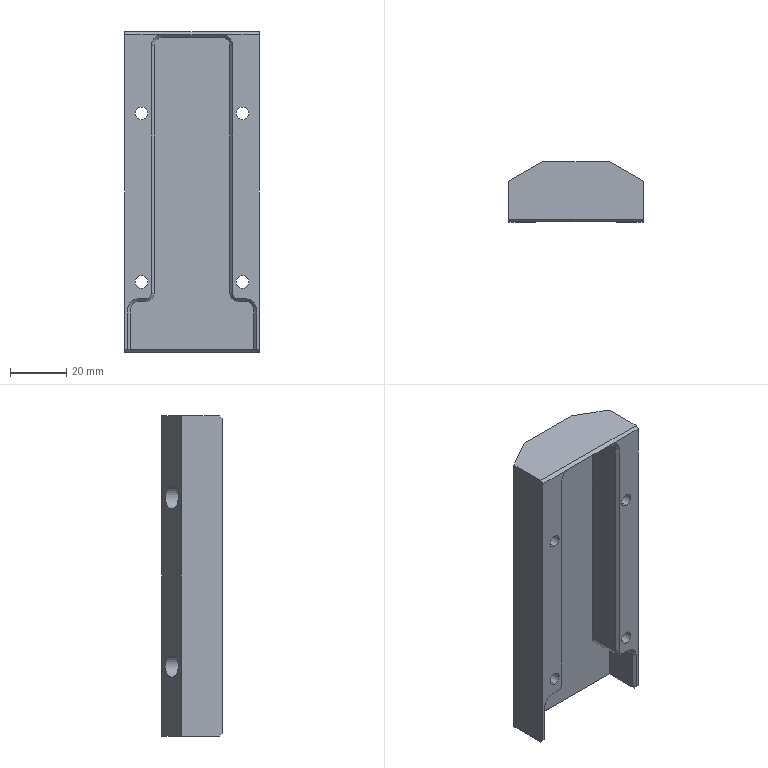CAM job | Mastercam | mm | 17 operations | part box 48 x 21.5 x 114
1. Contour (Ramp) | 9 - 10C 平底刀
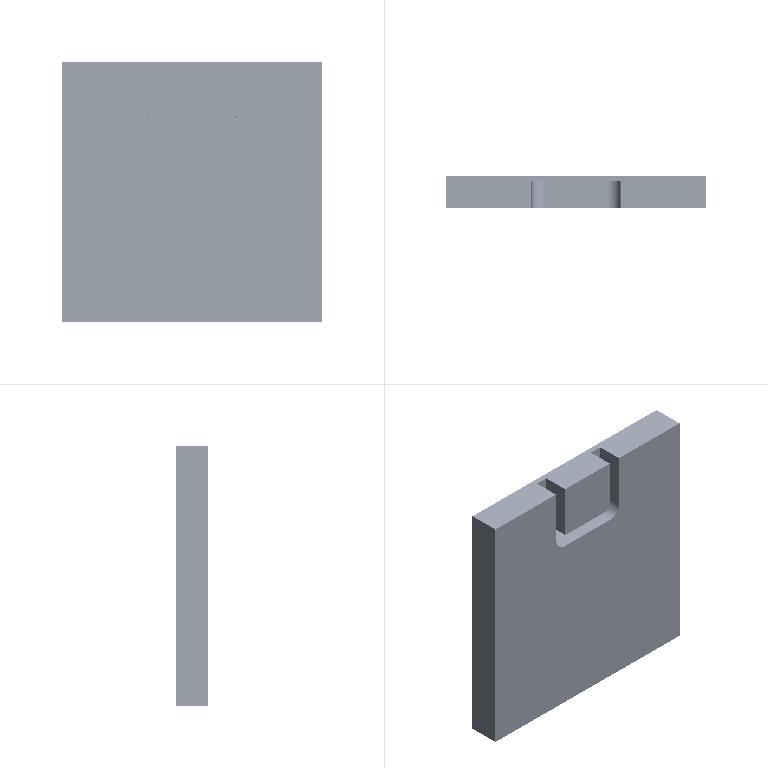2. Facing | 10 - 10J 平底刀
3. 2D High Speed (2D Dynamic Mill) | 6 - 6 平底刀
4. Drill/Counterbore | 2 - 4定位倒角
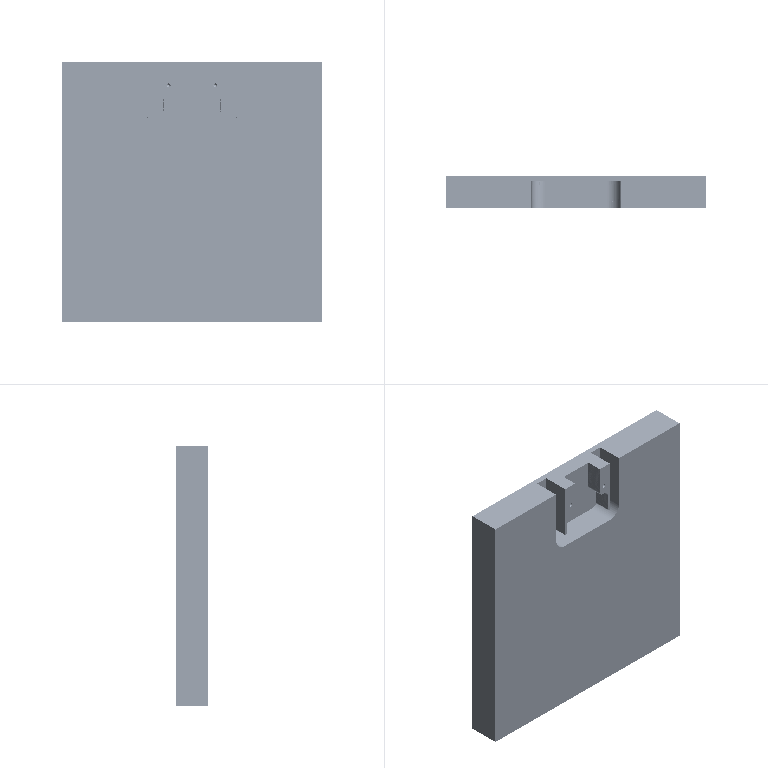5. Peck Drill | 18 - 4.5 钻头
6. Pocket (Open) | 8 - 6 J平底刀
7. Contour (2D) | 6 - 6 平底刀
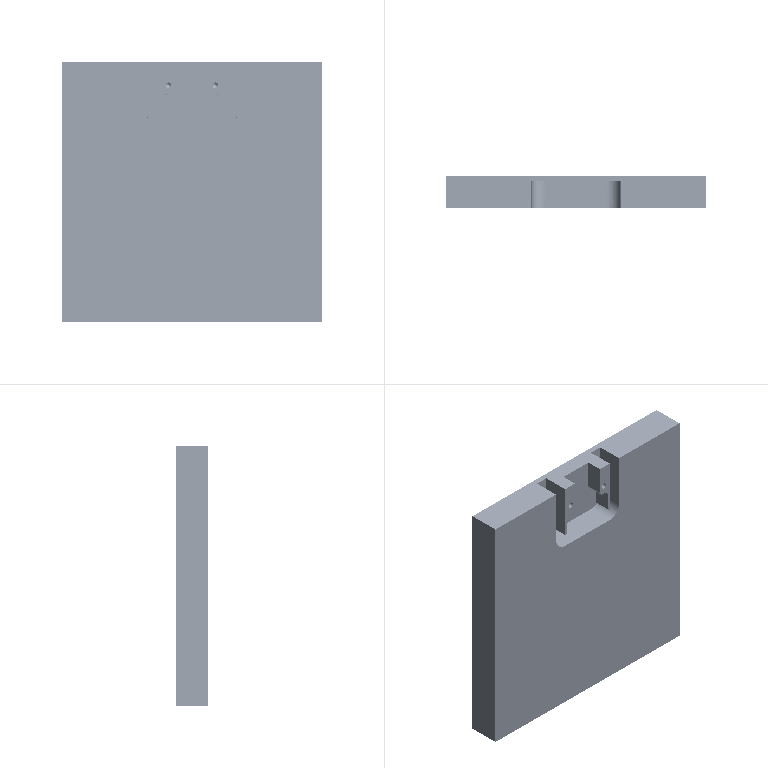8. Contour (2D chamfer) | 2 - 4定位倒角
9. Model Chamfer | 2 - 4定位倒角
10. Surface Finish Flowline | 20 - 4 -R0.5圆鼻铣刀
11. Contour (Ramp) | 9 - 10C 平底刀
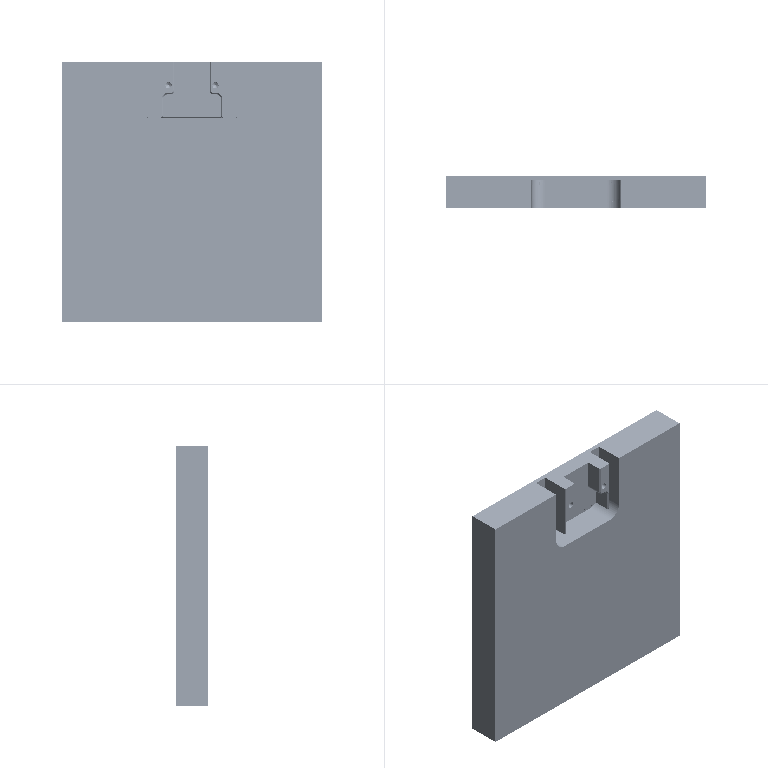12. Contour (2D) | 10 - 10J 平底刀
13. Facing | 1 - 50 J面铣
14. Helix Bore | 6 - 6 平底刀
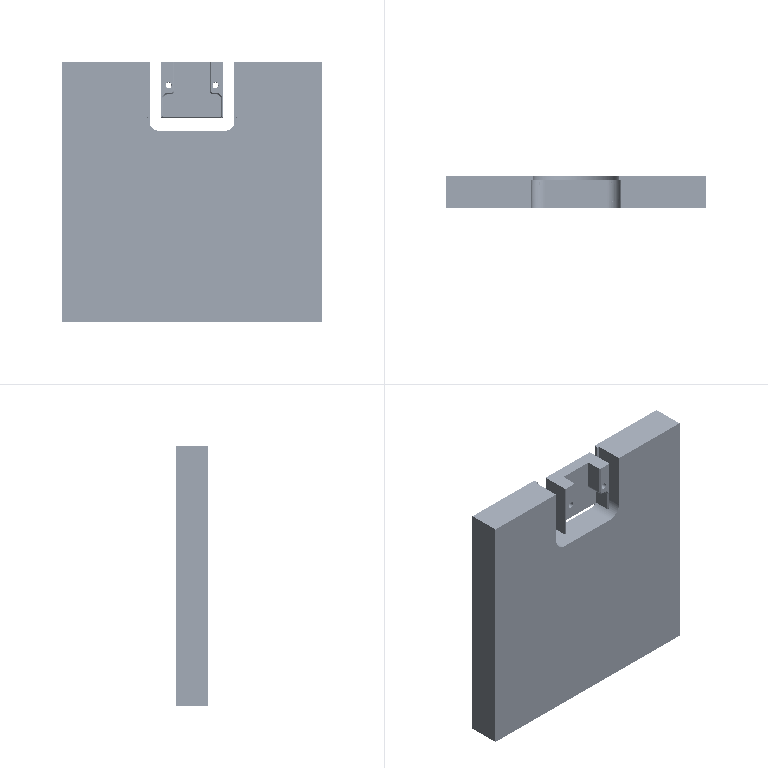15. Surface Finish Flowline | 3 - 10 -R1.0圆鼻铣刀
16. Deburr 5-axis Deburr 5-axis | 24 - 4 球刀
17. Contour (Ramp) | 9 - 10C 平底刀